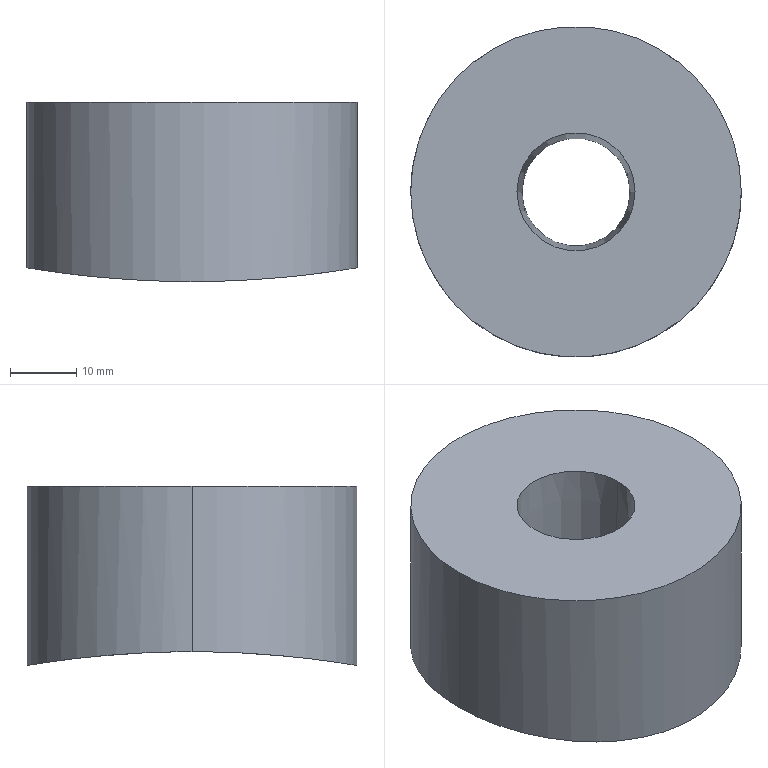Component | SolidWorks | JF21-80.1-1-3(_)-1-SOLID5-1 | 1 solid | 7 faces | box 50 x 50 x 27.1 mm | volume 44357 mm3 | cylinder 4 | cone 2 | plane 1 | commonest cylinder face diameters 300 x2 50 x2
STEP:
#1=COLOUR_RGB('',0.7922,0.8196,0.9333);
#2=FILL_AREA_STYLE_COLOUR('',#1);
#3=FILL_AREA_STYLE('',(#2));
#4=SURFACE_STYLE_FILL_AREA(#3);
#5=SURFACE_SIDE_STYLE('',(#4));
#6=SURFACE_STYLE_USAGE(.BOTH.,#5);
#7=PRESENTATION_STYLE_ASSIGNMENT((#6));
#8=CARTESIAN_POINT('',(9.252,-39.37,42.126));
#9=VERTEX_POINT('',#8);
#10=CARTESIAN_POINT('',(11.22,-39.37,42.126));
#11=VERTEX_POINT('',#10);
#12=CARTESIAN_POINT('',(9.252,-39.37,42.126));
#13=CARTESIAN_POINT('',(9.252,-39.435,42.126));
#14=CARTESIAN_POINT('',(9.258,-39.499,42.125));
#15=CARTESIAN_POINT('',(9.277,-39.594,42.122));
#16=CARTESIAN_POINT('',(9.285,-39.625,42.121));
#17=CARTESIAN_POINT('',(9.304,-39.687,42.118));
#18=CARTESIAN_POINT('',(9.315,-39.718,42.116));
#19=CARTESIAN_POINT('',(9.352,-39.807,42.11));
#20=CARTESIAN_POINT('',(9.382,-39.863,42.106));
#21=CARTESIAN_POINT('',(9.427,-39.93,42.099));
#22=CARTESIAN_POINT('',(9.436,-39.943,42.098));
#23=CARTESIAN_POINT('',(9.455,-39.969,42.096));
#24=CARTESIAN_POINT('',(9.465,-39.982,42.094));
#25=CARTESIAN_POINT('',(9.496,-40.02,42.09));
#26=CARTESIAN_POINT('',(9.518,-40.043,42.088));
#27=CARTESIAN_POINT('',(9.586,-40.111,42.079));
#28=CARTESIAN_POINT('',(9.635,-40.152,42.074));
#29=CARTESIAN_POINT('',(9.702,-40.197,42.068));
#30=CARTESIAN_POINT('',(9.716,-40.206,42.067));
#31=CARTESIAN_POINT('',(9.744,-40.222,42.064));
#32=CARTESIAN_POINT('',(9.758,-40.23,42.063));
#33=CARTESIAN_POINT('',(9.8,-40.253,42.06));
#34=CARTESIAN_POINT('',(9.829,-40.267,42.058));
#35=CARTESIAN_POINT('',(9.888,-40.291,42.054));
#36=CARTESIAN_POINT('',(9.919,-40.302,42.052));
#37=CARTESIAN_POINT('',(9.965,-40.316,42.05));
#38=CARTESIAN_POINT('',(9.98,-40.321,42.049));
#39=CARTESIAN_POINT('',(10.012,-40.329,42.048));
#40=CARTESIAN_POINT('',(10.028,-40.332,42.047));
#41=CARTESIAN_POINT('',(10.107,-40.348,42.044));
#42=CARTESIAN_POINT('',(10.171,-40.354,42.043));
#43=CARTESIAN_POINT('',(10.268,-40.354,42.043));
#44=CARTESIAN_POINT('',(10.3,-40.353,42.044));
#45=CARTESIAN_POINT('',(10.348,-40.348,42.044));
#46=CARTESIAN_POINT('',(10.365,-40.346,42.045));
#47=CARTESIAN_POINT('',(10.397,-40.341,42.046));
#48=CARTESIAN_POINT('',(10.412,-40.339,42.046));
#49=CARTESIAN_POINT('',(10.491,-40.323,42.049));
#50=CARTESIAN_POINT('',(10.553,-40.304,42.052));
#51=CARTESIAN_POINT('',(10.642,-40.267,42.057));
#52=CARTESIAN_POINT('',(10.672,-40.253,42.06));
#53=CARTESIAN_POINT('',(10.729,-40.223,42.064));
#54=CARTESIAN_POINT('',(10.756,-40.206,42.066));
#55=CARTESIAN_POINT('',(10.809,-40.171,42.071));
#56=CARTESIAN_POINT('',(10.835,-40.152,42.074));
#57=CARTESIAN_POINT('',(10.885,-40.111,42.079));
#58=CARTESIAN_POINT('',(10.909,-40.089,42.082));
#59=CARTESIAN_POINT('',(10.978,-40.021,42.09));
#60=CARTESIAN_POINT('',(11.018,-39.971,42.096));
#61=CARTESIAN_POINT('',(11.072,-39.891,42.103));
#62=CARTESIAN_POINT('',(11.088,-39.864,42.105));
#63=CARTESIAN_POINT('',(11.111,-39.821,42.109));
#64=CARTESIAN_POINT('',(11.119,-39.807,42.11));
#65=CARTESIAN_POINT('',(11.132,-39.777,42.112));
#66=CARTESIAN_POINT('',(11.139,-39.762,42.113));
#67=CARTESIAN_POINT('',(11.17,-39.688,42.118));
#68=CARTESIAN_POINT('',(11.189,-39.627,42.121));
#69=CARTESIAN_POINT('',(11.208,-39.532,42.124));
#70=CARTESIAN_POINT('',(11.212,-39.5,42.125));
#71=CARTESIAN_POINT('',(11.219,-39.435,42.126));
#72=CARTESIAN_POINT('',(11.22,-39.403,42.126));
#73=CARTESIAN_POINT('',(11.22,-39.37,42.126));
#74=B_SPLINE_CURVE_WITH_KNOTS('',3,(#12,#13,#14,#15,#16,#17,#18,#19,#20,#21,#22,#23,#24,#25,#26,#27,#28,#29,#30,#31,#32,#33,#34,#35,#36,#37,#38,#39,#40,#41,#42,#43,#44,#45,#46,#47,#48,#49,#50,#51,#52,#53,#54,#55,#56,#57,#58,#59,#60,#61,#62,#63,#64,#65,#66,#67,#68,#69,#70,#71,#72,#73),.UNSPECIFIED.,.F.,.F.,(4,2,2,2,2,2,2,2,2,2,2,2,2,2,2,2,2,2,2,2,2,2,2,2,2,2,2,2,2,2,4),(0.,0.004892,0.007339,0.009785,0.01468,0.0159,0.01712,0.01957,0.02446,0.02569,0.02691,0.02935,0.0318,0.03302,0.03425,0.03914,0.04159,0.04281,0.04403,0.04892,0.05137,0.05382,0.05626,0.05871,0.0636,0.06605,0.06727,0.06849,0.07339,0.07583,0.07828),.UNSPECIFIED.);
#75=EDGE_CURVE('',#9,#11,#74,.T.);
#76=ORIENTED_EDGE('',*,*,#75,.F.);
#77=CARTESIAN_POINT('',(9.915,-39.37,42.126));
#78=VERTEX_POINT('',#77);
#79=CARTESIAN_POINT('',(-15.748,-39.37,42.126));
#80=DIRECTION('',(1.,0.,0.));
#81=VECTOR('',#80,39.37);
#82=LINE('',#79,#81);
#83=EDGE_CURVE('',#9,#78,#82,.T.);
#84=ORIENTED_EDGE('',*,*,#83,.T.);
#85=CARTESIAN_POINT('',(10.557,-39.37,42.126));
#86=VERTEX_POINT('',#85);
#87=CARTESIAN_POINT('',(10.557,-39.37,42.126));
#88=CARTESIAN_POINT('',(10.557,-39.391,42.126));
#89=CARTESIAN_POINT('',(10.555,-39.412,42.126));
#90=CARTESIAN_POINT('',(10.549,-39.443,42.126));
#91=CARTESIAN_POINT('',(10.547,-39.453,42.125));
#92=CARTESIAN_POINT('',(10.541,-39.473,42.125));
#93=CARTESIAN_POINT('',(10.537,-39.483,42.125));
#94=CARTESIAN_POINT('',(10.525,-39.512,42.124));
#95=CARTESIAN_POINT('',(10.515,-39.531,42.124));
#96=CARTESIAN_POINT('',(10.492,-39.566,42.123));
#97=CARTESIAN_POINT('',(10.478,-39.582,42.122));
#98=CARTESIAN_POINT('',(10.448,-39.612,42.121));
#99=CARTESIAN_POINT('',(10.432,-39.625,42.12));
#100=CARTESIAN_POINT('',(10.406,-39.643,42.12));
#101=CARTESIAN_POINT('',(10.397,-39.648,42.119));
#102=CARTESIAN_POINT('',(10.378,-39.658,42.119));
#103=CARTESIAN_POINT('',(10.359,-39.667,42.119));
#104=CARTESIAN_POINT('',(10.34,-39.674,42.118));
#105=CARTESIAN_POINT('',(10.32,-39.68,42.118));
#106=CARTESIAN_POINT('',(10.309,-39.683,42.118));
#107=CARTESIAN_POINT('',(10.278,-39.689,42.117));
#108=CARTESIAN_POINT('',(10.257,-39.691,42.117));
#109=CARTESIAN_POINT('',(10.215,-39.691,42.117));
#110=CARTESIAN_POINT('',(10.194,-39.689,42.117));
#111=CARTESIAN_POINT('',(10.153,-39.681,42.118));
#112=CARTESIAN_POINT('',(10.133,-39.675,42.118));
#113=CARTESIAN_POINT('',(10.104,-39.663,42.119));
#114=CARTESIAN_POINT('',(10.094,-39.658,42.119));
#115=CARTESIAN_POINT('',(10.076,-39.648,42.119));
#116=CARTESIAN_POINT('',(10.067,-39.643,42.12));
#117=CARTESIAN_POINT('',(10.041,-39.625,42.12));
#118=CARTESIAN_POINT('',(10.024,-39.612,42.121));
#119=CARTESIAN_POINT('',(9.994,-39.582,42.122));
#120=CARTESIAN_POINT('',(9.981,-39.566,42.123));
#121=CARTESIAN_POINT('',(9.963,-39.54,42.124));
#122=CARTESIAN_POINT('',(9.958,-39.531,42.124));
#123=CARTESIAN_POINT('',(9.948,-39.512,42.124));
#124=CARTESIAN_POINT('',(9.944,-39.503,42.124));
#125=CARTESIAN_POINT('',(9.931,-39.474,42.125));
#126=CARTESIAN_POINT('',(9.925,-39.454,42.125));
#127=CARTESIAN_POINT('',(9.917,-39.413,42.126));
#128=CARTESIAN_POINT('',(9.915,-39.391,42.126));
#129=CARTESIAN_POINT('',(9.915,-39.37,42.126));
#130=B_SPLINE_CURVE_WITH_KNOTS('',3,(#87,#88,#89,#90,#91,#92,#93,#94,#95,#96,#97,#98,#99,#100,#101,#102,#103,#104,#105,#106,#107,#108,#109,#110,#111,#112,#113,#114,#115,#116,#117,#118,#119,#120,#121,#122,#123,#124,#125,#126,#127,#128,#129),.UNSPECIFIED.,.F.,.F.,(4,2,2,2,2,2,2,2,1,2,2,2,2,2,2,2,2,2,2,2,2,4),(0.,0.001594,0.002391,0.003187,0.004781,0.006375,0.007968,0.008765,0.009562,0.01036,0.01116,0.01275,0.01434,0.01594,0.01673,0.01753,0.01912,0.02072,0.02151,0.02231,0.02391,0.0255),.UNSPECIFIED.);
#131=EDGE_CURVE('',#86,#78,#130,.T.);
#132=ORIENTED_EDGE('',*,*,#131,.F.);
#133=CARTESIAN_POINT('',(-15.748,-39.37,42.126));
#134=DIRECTION('',(1.,0.,0.));
#135=VECTOR('',#134,39.37);
#136=LINE('',#133,#135);
#137=EDGE_CURVE('',#86,#11,#136,.T.);
#138=ORIENTED_EDGE('',*,*,#137,.T.);
#139=EDGE_LOOP('',(#76,#84,#132,#138));
#140=FACE_OUTER_BOUND('',#139,.T.);
#141=CARTESIAN_POINT('',(-15.748,-39.37,36.22));
#142=DIRECTION('',(1.,0.,0.));
#143=DIRECTION('',(0.,0.,1.));
#144=AXIS2_PLACEMENT_3D('',#141,#142,#143);
#145=CYLINDRICAL_SURFACE('',#144,5.906);
#146=ADVANCED_FACE('',(#140),#145,.F.);
#147=ORIENTED_EDGE('',*,*,#131,.T.);
#148=CARTESIAN_POINT('',(9.884,-39.37,43.11));
#149=VERTEX_POINT('',#148);
#150=CARTESIAN_POINT('',(9.884,-39.37,43.11));
#151=DIRECTION('',(-0.0312,0.,0.9995));
#152=VECTOR('',#151,39.37);
#153=LINE('',#150,#152);
#154=EDGE_CURVE('',#78,#149,#153,.T.);
#155=ORIENTED_EDGE('',*,*,#154,.T.);
#156=CARTESIAN_POINT('',(10.588,-39.37,43.11));
#157=VERTEX_POINT('',#156);
#158=CARTESIAN_POINT('',(10.236,-39.37,43.11));
#159=DIRECTION('',(0.,0.,1.));
#160=DIRECTION('',(1.,0.,0.));
#161=AXIS2_PLACEMENT_3D('',#158,#159,#160);
#162=CIRCLE('',#161,0.352);
#163=EDGE_CURVE('',#149,#157,#162,.T.);
#164=ORIENTED_EDGE('',*,*,#163,.T.);
#165=CARTESIAN_POINT('',(10.588,-39.37,43.11));
#166=DIRECTION('',(0.0312,0.,0.9995));
#167=VECTOR('',#166,39.37);
#168=LINE('',#165,#167);
#169=EDGE_CURVE('',#86,#157,#168,.T.);
#170=ORIENTED_EDGE('',*,*,#169,.F.);
#171=EDGE_LOOP('',(#147,#155,#164,#170));
#172=FACE_OUTER_BOUND('',#171,.T.);
#173=CARTESIAN_POINT('',(10.236,-39.37,43.11));
#174=DIRECTION('',(0.,0.,1.));
#175=DIRECTION('',(-1.,0.,0.));
#176=AXIS2_PLACEMENT_3D('',#173,#174,#175);
#177=CONICAL_SURFACE('',#176,0.352,0.03121);
#178=ADVANCED_FACE('',(#172),#177,.F.);
#179=CARTESIAN_POINT('',(11.22,-39.37,42.126));
#180=CARTESIAN_POINT('',(11.22,-39.305,42.126));
#181=CARTESIAN_POINT('',(11.214,-39.241,42.125));
#182=CARTESIAN_POINT('',(11.195,-39.146,42.122));
#183=CARTESIAN_POINT('',(11.187,-39.115,42.121));
#184=CARTESIAN_POINT('',(11.169,-39.053,42.118));
#185=CARTESIAN_POINT('',(11.158,-39.023,42.116));
#186=CARTESIAN_POINT('',(11.121,-38.933,42.11));
#187=CARTESIAN_POINT('',(11.09,-38.877,42.106));
#188=CARTESIAN_POINT('',(11.046,-38.81,42.099));
#189=CARTESIAN_POINT('',(11.036,-38.797,42.098));
#190=CARTESIAN_POINT('',(11.017,-38.771,42.096));
#191=CARTESIAN_POINT('',(11.007,-38.758,42.094));
#192=CARTESIAN_POINT('',(10.976,-38.721,42.09));
#193=CARTESIAN_POINT('',(10.955,-38.697,42.088));
#194=CARTESIAN_POINT('',(10.887,-38.629,42.079));
#195=CARTESIAN_POINT('',(10.837,-38.588,42.074));
#196=CARTESIAN_POINT('',(10.77,-38.543,42.068));
#197=CARTESIAN_POINT('',(10.756,-38.534,42.067));
#198=CARTESIAN_POINT('',(10.729,-38.518,42.064));
#199=CARTESIAN_POINT('',(10.715,-38.51,42.063));
#200=CARTESIAN_POINT('',(10.672,-38.487,42.06));
#201=CARTESIAN_POINT('',(10.643,-38.473,42.058));
#202=CARTESIAN_POINT('',(10.584,-38.449,42.054));
#203=CARTESIAN_POINT('',(10.554,-38.438,42.052));
#204=CARTESIAN_POINT('',(10.508,-38.424,42.05));
#205=CARTESIAN_POINT('',(10.492,-38.42,42.049));
#206=CARTESIAN_POINT('',(10.461,-38.412,42.048));
#207=CARTESIAN_POINT('',(10.445,-38.408,42.047));
#208=CARTESIAN_POINT('',(10.365,-38.392,42.044));
#209=CARTESIAN_POINT('',(10.301,-38.386,42.043));
#210=CARTESIAN_POINT('',(10.205,-38.386,42.043));
#211=CARTESIAN_POINT('',(10.173,-38.387,42.044));
#212=CARTESIAN_POINT('',(10.124,-38.392,42.044));
#213=CARTESIAN_POINT('',(10.108,-38.394,42.045));
#214=CARTESIAN_POINT('',(10.076,-38.399,42.046));
#215=CARTESIAN_POINT('',(10.06,-38.402,42.046));
#216=CARTESIAN_POINT('',(9.981,-38.417,42.049));
#217=CARTESIAN_POINT('',(9.92,-38.436,42.052));
#218=CARTESIAN_POINT('',(9.83,-38.473,42.057));
#219=CARTESIAN_POINT('',(9.801,-38.487,42.06));
#220=CARTESIAN_POINT('',(9.744,-38.517,42.064));
#221=CARTESIAN_POINT('',(9.716,-38.534,42.066));
#222=CARTESIAN_POINT('',(9.663,-38.569,42.071));
#223=CARTESIAN_POINT('',(9.637,-38.588,42.074));
#224=CARTESIAN_POINT('',(9.588,-38.629,42.079));
#225=CARTESIAN_POINT('',(9.564,-38.651,42.082));
#226=CARTESIAN_POINT('',(9.495,-38.719,42.09));
#227=CARTESIAN_POINT('',(9.454,-38.769,42.096));
#228=CARTESIAN_POINT('',(9.401,-38.849,42.103));
#229=CARTESIAN_POINT('',(9.384,-38.876,42.105));
#230=CARTESIAN_POINT('',(9.361,-38.919,42.109));
#231=CARTESIAN_POINT('',(9.354,-38.934,42.11));
#232=CARTESIAN_POINT('',(9.34,-38.963,42.112));
#233=CARTESIAN_POINT('',(9.333,-38.978,42.113));
#234=CARTESIAN_POINT('',(9.303,-39.052,42.118));
#235=CARTESIAN_POINT('',(9.284,-39.113,42.121));
#236=CARTESIAN_POINT('',(9.265,-39.208,42.124));
#237=CARTESIAN_POINT('',(9.26,-39.24,42.125));
#238=CARTESIAN_POINT('',(9.254,-39.305,42.126));
#239=CARTESIAN_POINT('',(9.252,-39.338,42.126));
#240=CARTESIAN_POINT('',(9.252,-39.37,42.126));
#241=B_SPLINE_CURVE_WITH_KNOTS('',3,(#179,#180,#181,#182,#183,#184,#185,#186,#187,#188,#189,#190,#191,#192,#193,#194,#195,#196,#197,#198,#199,#200,#201,#202,#203,#204,#205,#206,#207,#208,#209,#210,#211,#212,#213,#214,#215,#216,#217,#218,#219,#220,#221,#222,#223,#224,#225,#226,#227,#228,#229,#230,#231,#232,#233,#234,#235,#236,#237,#238,#239,#240),.UNSPECIFIED.,.F.,.F.,(4,2,2,2,2,2,2,2,2,2,2,2,2,2,2,2,2,2,2,2,2,2,2,2,2,2,2,2,2,2,4),(0.,0.004892,0.007339,0.009785,0.01468,0.0159,0.01712,0.01957,0.02446,0.02569,0.02691,0.02935,0.0318,0.03302,0.03425,0.03914,0.04159,0.04281,0.04403,0.04892,0.05137,0.05382,0.05626,0.05871,0.0636,0.06605,0.06727,0.06849,0.07339,0.07583,0.07828),.UNSPECIFIED.);
#242=EDGE_CURVE('',#11,#9,#241,.T.);
#243=ORIENTED_EDGE('',*,*,#242,.T.);
#244=CARTESIAN_POINT('',(9.252,-39.37,43.11));
#245=VERTEX_POINT('',#244);
#246=CARTESIAN_POINT('',(9.252,-39.37,41.929));
#247=DIRECTION('',(0.,0.,1.));
#248=VECTOR('',#247,39.37);
#249=LINE('',#246,#248);
#250=EDGE_CURVE('',#9,#245,#249,.T.);
#251=ORIENTED_EDGE('',*,*,#250,.T.);
#252=CARTESIAN_POINT('',(11.22,-39.37,43.11));
#253=VERTEX_POINT('',#252);
#254=CARTESIAN_POINT('',(10.236,-39.37,43.11));
#255=DIRECTION('',(0.,0.,1.));
#256=DIRECTION('',(1.,0.,0.));
#257=AXIS2_PLACEMENT_3D('',#254,#255,#256);
#258=CIRCLE('',#257,0.9843);
#259=EDGE_CURVE('',#253,#245,#258,.T.);
#260=ORIENTED_EDGE('',*,*,#259,.F.);
#261=CARTESIAN_POINT('',(11.22,-39.37,41.929));
#262=DIRECTION('',(0.,0.,1.));
#263=VECTOR('',#262,39.37);
#264=LINE('',#261,#263);
#265=EDGE_CURVE('',#11,#253,#264,.T.);
#266=ORIENTED_EDGE('',*,*,#265,.F.);
#267=EDGE_LOOP('',(#243,#251,#260,#266));
#268=FACE_OUTER_BOUND('',#267,.T.);
#269=CARTESIAN_POINT('',(10.236,-39.37,41.929));
#270=DIRECTION('',(0.,0.,1.));
#271=DIRECTION('',(-1.,0.,0.));
#272=AXIS2_PLACEMENT_3D('',#269,#270,#271);
#273=CYLINDRICAL_SURFACE('',#272,0.9843);
#274=ADVANCED_FACE('',(#268),#273,.T.);
#275=ORIENTED_EDGE('',*,*,#250,.F.);
#276=ORIENTED_EDGE('',*,*,#75,.T.);
#277=ORIENTED_EDGE('',*,*,#265,.T.);
#278=CARTESIAN_POINT('',(10.236,-39.37,43.11));
#279=DIRECTION('',(0.,0.,1.));
#280=DIRECTION('',(1.,0.,0.));
#281=AXIS2_PLACEMENT_3D('',#278,#279,#280);
#282=CIRCLE('',#281,0.9843);
#283=EDGE_CURVE('',#245,#253,#282,.T.);
#284=ORIENTED_EDGE('',*,*,#283,.F.);
#285=EDGE_LOOP('',(#275,#276,#277,#284));
#286=FACE_OUTER_BOUND('',#285,.T.);
#287=CARTESIAN_POINT('',(10.236,-39.37,41.929));
#288=DIRECTION('',(0.,0.,1.));
#289=DIRECTION('',(-1.,0.,0.));
#290=AXIS2_PLACEMENT_3D('',#287,#288,#289);
#291=CYLINDRICAL_SURFACE('',#290,0.9843);
#292=ADVANCED_FACE('',(#286),#291,.T.);
#293=CARTESIAN_POINT('',(10.236,-39.37,43.11));
#294=DIRECTION('',(0.,0.,1.));
#295=DIRECTION('',(1.,0.,0.));
#296=AXIS2_PLACEMENT_3D('',#293,#294,#295);
#297=CIRCLE('',#296,0.352);
#298=EDGE_CURVE('',#157,#149,#297,.T.);
#299=ORIENTED_EDGE('',*,*,#298,.F.);
#300=ORIENTED_EDGE('',*,*,#163,.F.);
#301=EDGE_LOOP('',(#299,#300));
#302=FACE_BOUND('',#301,.T.);
#303=ORIENTED_EDGE('',*,*,#259,.T.);
#304=ORIENTED_EDGE('',*,*,#283,.T.);
#305=EDGE_LOOP('',(#303,#304));
#306=FACE_OUTER_BOUND('',#305,.T.);
#307=CARTESIAN_POINT('',(10.236,-39.37,43.11));
#308=DIRECTION('',(0.,0.,1.));
#309=DIRECTION('',(-1.,0.,0.));
#310=AXIS2_PLACEMENT_3D('',#307,#308,#309);
#311=PLANE('',#310);
#312=ADVANCED_FACE('',(#302,#306),#311,.T.);
#313=ORIENTED_EDGE('',*,*,#83,.F.);
#314=ORIENTED_EDGE('',*,*,#242,.F.);
#315=ORIENTED_EDGE('',*,*,#137,.F.);
#316=CARTESIAN_POINT('',(9.915,-39.37,42.126));
#317=CARTESIAN_POINT('',(9.915,-39.349,42.126));
#318=CARTESIAN_POINT('',(9.917,-39.328,42.126));
#319=CARTESIAN_POINT('',(9.923,-39.297,42.126));
#320=CARTESIAN_POINT('',(9.926,-39.287,42.125));
#321=CARTESIAN_POINT('',(9.932,-39.267,42.125));
#322=CARTESIAN_POINT('',(9.935,-39.257,42.125));
#323=CARTESIAN_POINT('',(9.948,-39.228,42.124));
#324=CARTESIAN_POINT('',(9.957,-39.209,42.124));
#325=CARTESIAN_POINT('',(9.981,-39.174,42.123));
#326=CARTESIAN_POINT('',(9.994,-39.158,42.122));
#327=CARTESIAN_POINT('',(10.024,-39.128,42.121));
#328=CARTESIAN_POINT('',(10.04,-39.115,42.12));
#329=CARTESIAN_POINT('',(10.066,-39.097,42.12));
#330=CARTESIAN_POINT('',(10.076,-39.092,42.119));
#331=CARTESIAN_POINT('',(10.094,-39.082,42.119));
#332=CARTESIAN_POINT('',(10.113,-39.073,42.119));
#333=CARTESIAN_POINT('',(10.133,-39.066,42.118));
#334=CARTESIAN_POINT('',(10.153,-39.06,42.118));
#335=CARTESIAN_POINT('',(10.163,-39.057,42.118));
#336=CARTESIAN_POINT('',(10.194,-39.051,42.117));
#337=CARTESIAN_POINT('',(10.215,-39.049,42.117));
#338=CARTESIAN_POINT('',(10.257,-39.049,42.117));
#339=CARTESIAN_POINT('',(10.278,-39.051,42.117));
#340=CARTESIAN_POINT('',(10.319,-39.059,42.118));
#341=CARTESIAN_POINT('',(10.339,-39.065,42.118));
#342=CARTESIAN_POINT('',(10.369,-39.077,42.119));
#343=CARTESIAN_POINT('',(10.378,-39.082,42.119));
#344=CARTESIAN_POINT('',(10.397,-39.092,42.119));
#345=CARTESIAN_POINT('',(10.406,-39.097,42.12));
#346=CARTESIAN_POINT('',(10.432,-39.115,42.12));
#347=CARTESIAN_POINT('',(10.448,-39.128,42.121));
#348=CARTESIAN_POINT('',(10.478,-39.158,42.122));
#349=CARTESIAN_POINT('',(10.491,-39.174,42.123));
#350=CARTESIAN_POINT('',(10.509,-39.2,42.124));
#351=CARTESIAN_POINT('',(10.514,-39.209,42.124));
#352=CARTESIAN_POINT('',(10.524,-39.228,42.124));
#353=CARTESIAN_POINT('',(10.529,-39.237,42.124));
#354=CARTESIAN_POINT('',(10.541,-39.266,42.125));
#355=CARTESIAN_POINT('',(10.547,-39.286,42.125));
#356=CARTESIAN_POINT('',(10.555,-39.328,42.126));
#357=CARTESIAN_POINT('',(10.557,-39.349,42.126));
#358=CARTESIAN_POINT('',(10.557,-39.37,42.126));
#359=B_SPLINE_CURVE_WITH_KNOTS('',3,(#316,#317,#318,#319,#320,#321,#322,#323,#324,#325,#326,#327,#328,#329,#330,#331,#332,#333,#334,#335,#336,#337,#338,#339,#340,#341,#342,#343,#344,#345,#346,#347,#348,#349,#350,#351,#352,#353,#354,#355,#356,#357,#358),.UNSPECIFIED.,.F.,.F.,(4,2,2,2,2,2,2,2,1,2,2,2,2,2,2,2,2,2,2,2,2,4),(0.,0.001594,0.002391,0.003187,0.004781,0.006375,0.007968,0.008765,0.009562,0.01036,0.01116,0.01275,0.01434,0.01594,0.01673,0.01753,0.01912,0.02072,0.02151,0.02231,0.02391,0.0255),.UNSPECIFIED.);
#360=EDGE_CURVE('',#78,#86,#359,.T.);
#361=ORIENTED_EDGE('',*,*,#360,.F.);
#362=EDGE_LOOP('',(#313,#314,#315,#361));
#363=FACE_OUTER_BOUND('',#362,.T.);
#364=CARTESIAN_POINT('',(-15.748,-39.37,36.22));
#365=DIRECTION('',(1.,0.,0.));
#366=DIRECTION('',(0.,0.,1.));
#367=AXIS2_PLACEMENT_3D('',#364,#365,#366);
#368=CYLINDRICAL_SURFACE('',#367,5.906);
#369=ADVANCED_FACE('',(#363),#368,.F.);
#370=ORIENTED_EDGE('',*,*,#154,.F.);
#371=ORIENTED_EDGE('',*,*,#360,.T.);
#372=ORIENTED_EDGE('',*,*,#169,.T.);
#373=ORIENTED_EDGE('',*,*,#298,.T.);
#374=EDGE_LOOP('',(#370,#371,#372,#373));
#375=FACE_OUTER_BOUND('',#374,.T.);
#376=CARTESIAN_POINT('',(10.236,-39.37,43.11));
#377=DIRECTION('',(0.,0.,1.));
#378=DIRECTION('',(-1.,0.,0.));
#379=AXIS2_PLACEMENT_3D('',#376,#377,#378);
#380=CONICAL_SURFACE('',#379,0.352,0.03121);
#381=ADVANCED_FACE('',(#375),#380,.F.);
#382=CLOSED_SHELL('',(#146,#178,#274,#292,#312,#369,#381));
#383=MANIFOLD_SOLID_BREP('',#382);
#384=STYLED_ITEM('',(#7),#383);
#385=(LENGTH_UNIT()NAMED_UNIT(*)SI_UNIT($,.METRE.));
#386=LENGTH_MEASURE_WITH_UNIT(LENGTH_MEASURE(0.0254),#385);
#387=DIMENSIONAL_EXPONENTS(1.,0.,0.,0.,0.,0.,0.);
#388=(CONVERSION_BASED_UNIT('',#386)LENGTH_UNIT()NAMED_UNIT(#387));
#389=UNCERTAINTY_MEASURE_WITH_UNIT(LENGTH_MEASURE(0.00001),#388,'','');
#390=(NAMED_UNIT(*)PLANE_ANGLE_UNIT()SI_UNIT($,.RADIAN.));
#391=(NAMED_UNIT(*)SI_UNIT($,.STERADIAN.)SOLID_ANGLE_UNIT());
#392=(GEOMETRIC_REPRESENTATION_CONTEXT(3)GLOBAL_UNCERTAINTY_ASSIGNED_CONTEXT((#389))GLOBAL_UNIT_ASSIGNED_CONTEXT((#388,#390,#391))REPRESENTATION_CONTEXT('',''));
#393=MECHANICAL_DESIGN_GEOMETRIC_PRESENTATION_REPRESENTATION('',(#384),#392);
#394=PRESENTATION_LAYER_ASSIGNMENT('','',(#384));
#395=CARTESIAN_POINT('',(0.,0.,0.));
#396=DIRECTION('',(0.,0.,1.));
#397=DIRECTION('',(1.,0.,0.));
#398=AXIS2_PLACEMENT_3D('',#395,#396,#397);
#399=(LENGTH_UNIT()NAMED_UNIT(*)SI_UNIT($,.METRE.));
#400=LENGTH_MEASURE_WITH_UNIT(LENGTH_MEASURE(0.0254),#399);
#401=DIMENSIONAL_EXPONENTS(1.,0.,0.,0.,0.,0.,0.);
#402=(CONVERSION_BASED_UNIT('',#400)LENGTH_UNIT()NAMED_UNIT(#401));
#403=UNCERTAINTY_MEASURE_WITH_UNIT(LENGTH_MEASURE(0.00001),#402,'','');
#404=(NAMED_UNIT(*)PLANE_ANGLE_UNIT()SI_UNIT($,.RADIAN.));
#405=(NAMED_UNIT(*)SI_UNIT($,.STERADIAN.)SOLID_ANGLE_UNIT());
#406=(GEOMETRIC_REPRESENTATION_CONTEXT(3)GLOBAL_UNCERTAINTY_ASSIGNED_CONTEXT((#403))GLOBAL_UNIT_ASSIGNED_CONTEXT((#402,#404,#405))REPRESENTATION_CONTEXT('',''));
#407=ADVANCED_BREP_SHAPE_REPRESENTATION('',(#383,#398),#406);